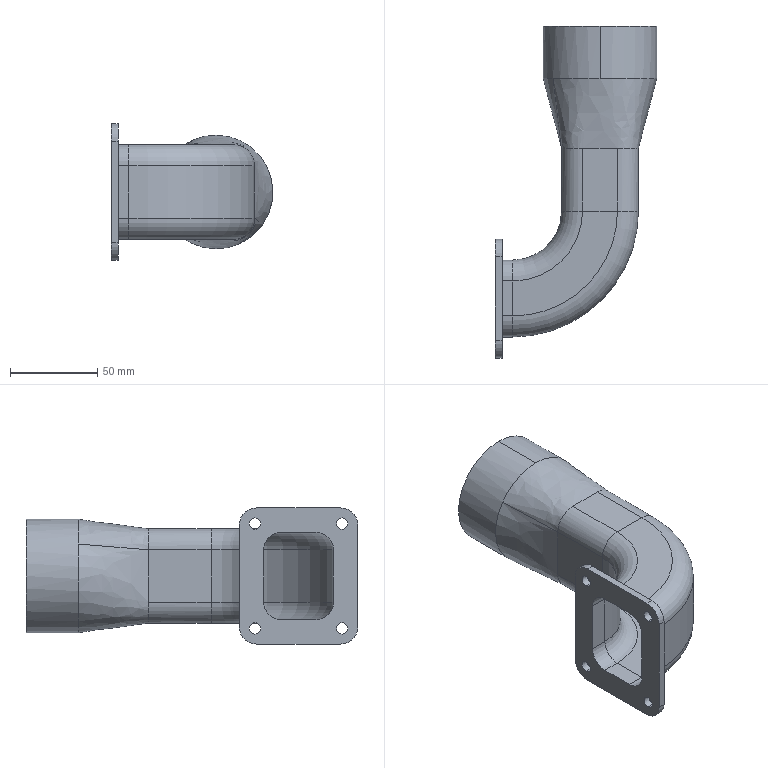Component | SolidWorks | SeedingAssemblyA-1_SeedInlet-1 | 1 solid | 75 faces | volume 79908 mm3 | cylinder 36 | plane 27 | torus 8 | spline 4 | commonest cylinder face diameters 20 x12 6.5 x8 24 x8 61 x2 65 x2 56 x1 144 x1 60 x1